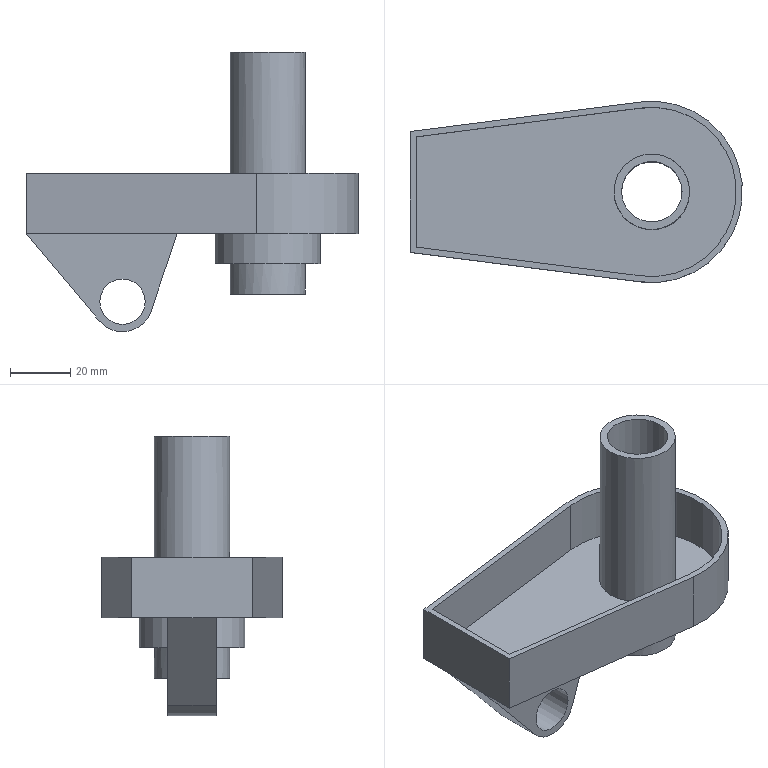Component | NX | LEFT_RIGHT_BRACKET | 1 solid | 24 faces | volume 52179 mm3 | plane 16 | cylinder 8 | commonest cylinder face diameters 20 x2 25 x2 60 x1 56 x1 15 x1 35 x1